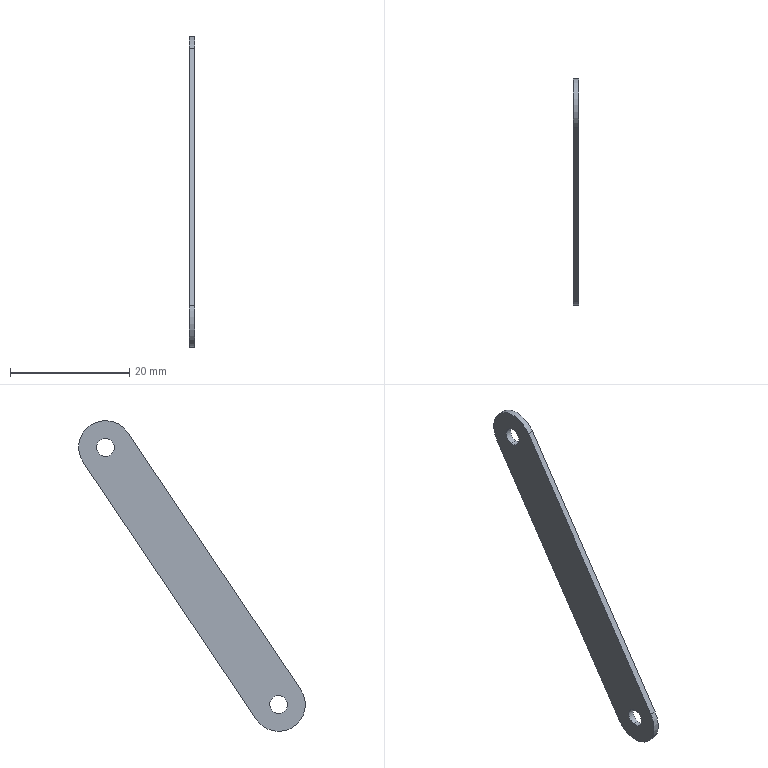Component | SolidWorks | Part12-2 | 1 solid | 11 faces | box 1 x 38.06 x 52.17 mm | volume 518 mm3 | cylinder 7 | plane 4 | commonest cylinder face diameters 3 x4 9 x3
build123d program:
from build123d import *

# Parameters (mm, degrees)
BOSS_EXTRUDE1_DEPTH = 1
BOSS_EXTRUDE2_START = -1
BOSS_EXTRUDE2_DEPTH = 1


with BuildPart() as part:
    # Sketch1 → Boss-Extrude1 (new body)
    with BuildSketch(Plane.XY):
        with BuildLine():
            Line((6.19, 34.803), (42.061, 72.502))
            ThreePointArc((42.061, 72.502), (48.423, 72.66), (48.581, 66.298))
            Line((48.581, 66.298), (12.71, 28.599))
            ThreePointArc((12.71, 28.599), (6.348, 28.441), (6.19, 34.803))
        make_face()
        with BuildLine():
            Line((8.363, 32.735), (44.235, 70.434))
            ThreePointArc((44.235, 70.434), (46.355, 70.487), (46.408, 68.366))
            Line((46.408, 68.366), (10.536, 30.667))
            ThreePointArc((10.536, 30.667), (8.416, 30.614), (8.363, 32.735))
        make_face(mode=Mode.SUBTRACT)
    extrude(amount=BOSS_EXTRUDE1_DEPTH)

    # Sketch2 → Boss-Extrude2 (add)
    with BuildSketch(Plane.XY.offset(1).offset(BOSS_EXTRUDE2_START)):
        with BuildLine():
            Line((10.536, 30.667), (46.408, 68.366))
            ThreePointArc((46.408, 68.366), (44.287, 68.314), (44.235, 70.434))
            Line((44.235, 70.434), (8.363, 32.735))
            ThreePointArc((8.363, 32.735), (10.484, 32.788), (10.536, 30.667))
        make_face()
    extrude(amount=BOSS_EXTRUDE2_DEPTH)


solid = part.part

# Placed as in the assembly
solid = solid.moved(Location((89.229, 6.521, -1.578), (12.475, -90, 0)))
STEP:
#1=COLOUR_RGB('',0.7922,0.8196,0.9333);
#2=FILL_AREA_STYLE_COLOUR('',#1);
#3=FILL_AREA_STYLE('',(#2));
#4=SURFACE_STYLE_FILL_AREA(#3);
#5=SURFACE_SIDE_STYLE('',(#4));
#6=SURFACE_STYLE_USAGE(.BOTH.,#5);
#7=PRESENTATION_STYLE_ASSIGNMENT((#6));
#8=CARTESIAN_POINT('',(3.474,2.552,2.213));
#9=VERTEX_POINT('',#8);
#10=CARTESIAN_POINT('',(3.474,2.526,2.328));
#11=VERTEX_POINT('',#10);
#12=CARTESIAN_POINT('',(3.474,2.539,2.27));
#13=DIRECTION('',(-1.,0.,0.));
#14=DIRECTION('',(0.,-0.216,0.9764));
#15=AXIS2_PLACEMENT_3D('',#12,#13,#14);
#16=CIRCLE('',#15,0.05906);
#17=EDGE_CURVE('',#9,#11,#16,.T.);
#18=ORIENTED_EDGE('',*,*,#17,.T.);
#19=CARTESIAN_POINT('',(3.513,2.526,2.328));
#20=VERTEX_POINT('',#19);
#21=CARTESIAN_POINT('',(3.474,2.526,2.328));
#22=DIRECTION('',(1.,-0.,-0.));
#23=VECTOR('',#22,39.37);
#24=LINE('',#21,#23);
#25=EDGE_CURVE('',#11,#20,#24,.T.);
#26=ORIENTED_EDGE('',*,*,#25,.T.);
#27=CARTESIAN_POINT('',(3.513,2.552,2.213));
#28=VERTEX_POINT('',#27);
#29=CARTESIAN_POINT('',(3.513,2.539,2.27));
#30=DIRECTION('',(-1.,0.,0.));
#31=DIRECTION('',(0.,-0.216,0.9764));
#32=AXIS2_PLACEMENT_3D('',#29,#30,#31);
#33=CIRCLE('',#32,0.05906);
#34=EDGE_CURVE('',#28,#20,#33,.T.);
#35=ORIENTED_EDGE('',*,*,#34,.F.);
#36=CARTESIAN_POINT('',(3.474,2.552,2.213));
#37=DIRECTION('',(1.,-0.,-0.));
#38=VECTOR('',#37,39.37);
#39=LINE('',#36,#38);
#40=EDGE_CURVE('',#9,#28,#39,.T.);
#41=ORIENTED_EDGE('',*,*,#40,.F.);
#42=EDGE_LOOP('',(#18,#26,#35,#41));
#43=FACE_OUTER_BOUND('',#42,.T.);
#44=CARTESIAN_POINT('',(3.474,2.539,2.27));
#45=DIRECTION('',(1.,-0.,-0.));
#46=DIRECTION('',(0.,0.216,-0.9764));
#47=AXIS2_PLACEMENT_3D('',#44,#45,#46);
#48=CYLINDRICAL_SURFACE('',#47,0.05906);
#49=ADVANCED_FACE('',(#43),#48,.F.);
#50=CARTESIAN_POINT('',(3.474,1.408,0.5131));
#51=VERTEX_POINT('',#50);
#52=CARTESIAN_POINT('',(3.474,1.382,0.6284));
#53=VERTEX_POINT('',#52);
#54=CARTESIAN_POINT('',(3.474,1.395,0.5707));
#55=DIRECTION('',(-1.,0.,0.));
#56=DIRECTION('',(0.,-0.216,0.9764));
#57=AXIS2_PLACEMENT_3D('',#54,#55,#56);
#58=CIRCLE('',#57,0.05906);
#59=EDGE_CURVE('',#51,#53,#58,.T.);
#60=ORIENTED_EDGE('',*,*,#59,.T.);
#61=CARTESIAN_POINT('',(3.513,1.382,0.6284));
#62=VERTEX_POINT('',#61);
#63=CARTESIAN_POINT('',(3.474,1.382,0.6284));
#64=DIRECTION('',(1.,-0.,-0.));
#65=VECTOR('',#64,39.37);
#66=LINE('',#63,#65);
#67=EDGE_CURVE('',#53,#62,#66,.T.);
#68=ORIENTED_EDGE('',*,*,#67,.T.);
#69=CARTESIAN_POINT('',(3.513,1.408,0.5131));
#70=VERTEX_POINT('',#69);
#71=CARTESIAN_POINT('',(3.513,1.395,0.5707));
#72=DIRECTION('',(-1.,0.,0.));
#73=DIRECTION('',(0.,-0.216,0.9764));
#74=AXIS2_PLACEMENT_3D('',#71,#72,#73);
#75=CIRCLE('',#74,0.05906);
#76=EDGE_CURVE('',#70,#62,#75,.T.);
#77=ORIENTED_EDGE('',*,*,#76,.F.);
#78=CARTESIAN_POINT('',(3.474,1.408,0.5131));
#79=DIRECTION('',(1.,-0.,-0.));
#80=VECTOR('',#79,39.37);
#81=LINE('',#78,#80);
#82=EDGE_CURVE('',#51,#70,#81,.T.);
#83=ORIENTED_EDGE('',*,*,#82,.F.);
#84=EDGE_LOOP('',(#60,#68,#77,#83));
#85=FACE_OUTER_BOUND('',#84,.T.);
#86=CARTESIAN_POINT('',(3.474,1.395,0.5707));
#87=DIRECTION('',(1.,-0.,-0.));
#88=DIRECTION('',(0.,0.216,-0.9764));
#89=AXIS2_PLACEMENT_3D('',#86,#87,#88);
#90=CYLINDRICAL_SURFACE('',#89,0.05906);
#91=ADVANCED_FACE('',(#85),#90,.F.);
#92=CARTESIAN_POINT('',(3.474,1.433,0.3978));
#93=VERTEX_POINT('',#92);
#94=CARTESIAN_POINT('',(3.474,1.248,0.6697));
#95=VERTEX_POINT('',#94);
#96=CARTESIAN_POINT('',(3.474,1.395,0.5707));
#97=DIRECTION('',(-1.,0.,0.));
#98=DIRECTION('',(0.,-0.216,0.9764));
#99=AXIS2_PLACEMENT_3D('',#96,#97,#98);
#100=CIRCLE('',#99,0.1772);
#101=EDGE_CURVE('',#93,#95,#100,.T.);
#102=ORIENTED_EDGE('',*,*,#101,.F.);
#103=CARTESIAN_POINT('',(3.513,1.433,0.3978));
#104=VERTEX_POINT('',#103);
#105=CARTESIAN_POINT('',(3.474,1.433,0.3978));
#106=DIRECTION('',(1.,-0.,-0.));
#107=VECTOR('',#106,39.37);
#108=LINE('',#105,#107);
#109=EDGE_CURVE('',#93,#104,#108,.T.);
#110=ORIENTED_EDGE('',*,*,#109,.T.);
#111=CARTESIAN_POINT('',(3.513,1.248,0.6697));
#112=VERTEX_POINT('',#111);
#113=CARTESIAN_POINT('',(3.513,1.395,0.5707));
#114=DIRECTION('',(-1.,0.,0.));
#115=DIRECTION('',(0.,-0.216,0.9764));
#116=AXIS2_PLACEMENT_3D('',#113,#114,#115);
#117=CIRCLE('',#116,0.1772);
#118=EDGE_CURVE('',#104,#112,#117,.T.);
#119=ORIENTED_EDGE('',*,*,#118,.T.);
#120=CARTESIAN_POINT('',(3.474,1.248,0.6697));
#121=DIRECTION('',(1.,-0.,-0.));
#122=VECTOR('',#121,39.37);
#123=LINE('',#120,#122);
#124=EDGE_CURVE('',#95,#112,#123,.T.);
#125=ORIENTED_EDGE('',*,*,#124,.F.);
#126=EDGE_LOOP('',(#102,#110,#119,#125));
#127=FACE_OUTER_BOUND('',#126,.T.);
#128=CARTESIAN_POINT('',(3.474,1.395,0.5707));
#129=DIRECTION('',(1.,-0.,-0.));
#130=DIRECTION('',(0.,0.216,-0.9764));
#131=AXIS2_PLACEMENT_3D('',#128,#129,#130);
#132=CYLINDRICAL_SURFACE('',#131,0.1772);
#133=ADVANCED_FACE('',(#127),#132,.T.);
#134=ORIENTED_EDGE('',*,*,#17,.F.);
#135=CARTESIAN_POINT('',(3.474,2.539,2.27));
#136=DIRECTION('',(-1.,0.,0.));
#137=DIRECTION('',(0.,-0.216,0.9764));
#138=AXIS2_PLACEMENT_3D('',#135,#136,#137);
#139=CIRCLE('',#138,0.05906);
#140=EDGE_CURVE('',#11,#9,#139,.T.);
#141=ORIENTED_EDGE('',*,*,#140,.F.);
#142=EDGE_LOOP('',(#134,#141));
#143=FACE_BOUND('',#142,.T.);
#144=CARTESIAN_POINT('',(3.474,1.542,0.4718));
#145=VERTEX_POINT('',#144);
#146=CARTESIAN_POINT('',(3.474,1.395,0.5707));
#147=DIRECTION('',(-1.,0.,0.));
#148=DIRECTION('',(0.,-0.216,0.9764));
#149=AXIS2_PLACEMENT_3D('',#146,#147,#148);
#150=CIRCLE('',#149,0.1772);
#151=EDGE_CURVE('',#145,#93,#150,.T.);
#152=ORIENTED_EDGE('',*,*,#151,.T.);
#153=ORIENTED_EDGE('',*,*,#101,.T.);
#154=CARTESIAN_POINT('',(3.474,2.392,2.369));
#155=VERTEX_POINT('',#154);
#156=CARTESIAN_POINT('',(3.474,1.248,0.6697));
#157=DIRECTION('',(0.,0.5584,0.8295));
#158=VECTOR('',#157,39.37);
#159=LINE('',#156,#158);
#160=EDGE_CURVE('',#95,#155,#159,.T.);
#161=ORIENTED_EDGE('',*,*,#160,.T.);
#162=CARTESIAN_POINT('',(3.474,2.686,2.171));
#163=VERTEX_POINT('',#162);
#164=CARTESIAN_POINT('',(3.474,2.539,2.27));
#165=DIRECTION('',(-1.,0.,0.));
#166=DIRECTION('',(0.,-0.216,0.9764));
#167=AXIS2_PLACEMENT_3D('',#164,#165,#166);
#168=CIRCLE('',#167,0.1772);
#169=EDGE_CURVE('',#155,#163,#168,.T.);
#170=ORIENTED_EDGE('',*,*,#169,.T.);
#171=CARTESIAN_POINT('',(3.474,1.542,0.4718));
#172=DIRECTION('',(-0.,-0.5584,-0.8295));
#173=VECTOR('',#172,39.37);
#174=LINE('',#171,#173);
#175=EDGE_CURVE('',#163,#145,#174,.T.);
#176=ORIENTED_EDGE('',*,*,#175,.T.);
#177=EDGE_LOOP('',(#152,#153,#161,#170,#176));
#178=FACE_OUTER_BOUND('',#177,.T.);
#179=ORIENTED_EDGE('',*,*,#59,.F.);
#180=CARTESIAN_POINT('',(3.474,1.395,0.5707));
#181=DIRECTION('',(-1.,0.,0.));
#182=DIRECTION('',(0.,-0.216,0.9764));
#183=AXIS2_PLACEMENT_3D('',#180,#181,#182);
#184=CIRCLE('',#183,0.05906);
#185=EDGE_CURVE('',#53,#51,#184,.T.);
#186=ORIENTED_EDGE('',*,*,#185,.F.);
#187=EDGE_LOOP('',(#179,#186));
#188=FACE_BOUND('',#187,.T.);
#189=CARTESIAN_POINT('',(3.474,1.395,0.5707));
#190=DIRECTION('',(-1.,0.,0.));
#191=DIRECTION('',(0.,-0.216,0.9764));
#192=AXIS2_PLACEMENT_3D('',#189,#190,#191);
#193=PLANE('',#192);
#194=ADVANCED_FACE('',(#143,#178,#188),#193,.T.);
#195=ORIENTED_EDGE('',*,*,#34,.T.);
#196=CARTESIAN_POINT('',(3.513,2.539,2.27));
#197=DIRECTION('',(-1.,0.,0.));
#198=DIRECTION('',(0.,-0.216,0.9764));
#199=AXIS2_PLACEMENT_3D('',#196,#197,#198);
#200=CIRCLE('',#199,0.05906);
#201=EDGE_CURVE('',#20,#28,#200,.T.);
#202=ORIENTED_EDGE('',*,*,#201,.T.);
#203=EDGE_LOOP('',(#195,#202));
#204=FACE_BOUND('',#203,.T.);
#205=CARTESIAN_POINT('',(3.513,1.542,0.4718));
#206=VERTEX_POINT('',#205);
#207=CARTESIAN_POINT('',(3.513,1.395,0.5707));
#208=DIRECTION('',(-1.,0.,0.));
#209=DIRECTION('',(0.,-0.216,0.9764));
#210=AXIS2_PLACEMENT_3D('',#207,#208,#209);
#211=CIRCLE('',#210,0.1772);
#212=EDGE_CURVE('',#206,#104,#211,.T.);
#213=ORIENTED_EDGE('',*,*,#212,.F.);
#214=CARTESIAN_POINT('',(3.513,2.686,2.171));
#215=VERTEX_POINT('',#214);
#216=CARTESIAN_POINT('',(3.513,1.542,0.4718));
#217=DIRECTION('',(-0.,-0.5584,-0.8295));
#218=VECTOR('',#217,39.37);
#219=LINE('',#216,#218);
#220=EDGE_CURVE('',#215,#206,#219,.T.);
#221=ORIENTED_EDGE('',*,*,#220,.F.);
#222=CARTESIAN_POINT('',(3.513,2.392,2.369));
#223=VERTEX_POINT('',#222);
#224=CARTESIAN_POINT('',(3.513,2.539,2.27));
#225=DIRECTION('',(-1.,0.,0.));
#226=DIRECTION('',(0.,-0.216,0.9764));
#227=AXIS2_PLACEMENT_3D('',#224,#225,#226);
#228=CIRCLE('',#227,0.1772);
#229=EDGE_CURVE('',#223,#215,#228,.T.);
#230=ORIENTED_EDGE('',*,*,#229,.F.);
#231=CARTESIAN_POINT('',(3.513,1.248,0.6697));
#232=DIRECTION('',(0.,0.5584,0.8295));
#233=VECTOR('',#232,39.37);
#234=LINE('',#231,#233);
#235=EDGE_CURVE('',#112,#223,#234,.T.);
#236=ORIENTED_EDGE('',*,*,#235,.F.);
#237=ORIENTED_EDGE('',*,*,#118,.F.);
#238=EDGE_LOOP('',(#213,#221,#230,#236,#237));
#239=FACE_OUTER_BOUND('',#238,.T.);
#240=ORIENTED_EDGE('',*,*,#76,.T.);
#241=CARTESIAN_POINT('',(3.513,1.395,0.5707));
#242=DIRECTION('',(-1.,0.,0.));
#243=DIRECTION('',(0.,-0.216,0.9764));
#244=AXIS2_PLACEMENT_3D('',#241,#242,#243);
#245=CIRCLE('',#244,0.05906);
#246=EDGE_CURVE('',#62,#70,#245,.T.);
#247=ORIENTED_EDGE('',*,*,#246,.T.);
#248=EDGE_LOOP('',(#240,#247));
#249=FACE_BOUND('',#248,.T.);
#250=CARTESIAN_POINT('',(3.513,1.395,0.5707));
#251=DIRECTION('',(-1.,0.,0.));
#252=DIRECTION('',(0.,-0.216,0.9764));
#253=AXIS2_PLACEMENT_3D('',#250,#251,#252);
#254=PLANE('',#253);
#255=ADVANCED_FACE('',(#204,#239,#249),#254,.F.);
#256=ORIENTED_EDGE('',*,*,#109,.F.);
#257=ORIENTED_EDGE('',*,*,#151,.F.);
#258=CARTESIAN_POINT('',(3.474,1.542,0.4718));
#259=DIRECTION('',(1.,-0.,-0.));
#260=VECTOR('',#259,39.37);
#261=LINE('',#258,#260);
#262=EDGE_CURVE('',#145,#206,#261,.T.);
#263=ORIENTED_EDGE('',*,*,#262,.T.);
#264=ORIENTED_EDGE('',*,*,#212,.T.);
#265=EDGE_LOOP('',(#256,#257,#263,#264));
#266=FACE_OUTER_BOUND('',#265,.T.);
#267=CARTESIAN_POINT('',(3.474,1.395,0.5707));
#268=DIRECTION('',(1.,-0.,-0.));
#269=DIRECTION('',(0.,0.216,-0.9764));
#270=AXIS2_PLACEMENT_3D('',#267,#268,#269);
#271=CYLINDRICAL_SURFACE('',#270,0.1772);
#272=ADVANCED_FACE('',(#266),#271,.T.);
#273=ORIENTED_EDGE('',*,*,#235,.T.);
#274=CARTESIAN_POINT('',(3.474,2.392,2.369));
#275=DIRECTION('',(1.,-0.,-0.));
#276=VECTOR('',#275,39.37);
#277=LINE('',#274,#276);
#278=EDGE_CURVE('',#155,#223,#277,.T.);
#279=ORIENTED_EDGE('',*,*,#278,.F.);
#280=ORIENTED_EDGE('',*,*,#160,.F.);
#281=ORIENTED_EDGE('',*,*,#124,.T.);
#282=EDGE_LOOP('',(#273,#279,#280,#281));
#283=FACE_OUTER_BOUND('',#282,.T.);
#284=CARTESIAN_POINT('',(3.474,1.248,0.6697));
#285=DIRECTION('',(0.,0.8295,-0.5584));
#286=DIRECTION('',(-0.,-0.5584,-0.8295));
#287=AXIS2_PLACEMENT_3D('',#284,#285,#286);
#288=PLANE('',#287);
#289=ADVANCED_FACE('',(#283),#288,.F.);
#290=ORIENTED_EDGE('',*,*,#229,.T.);
#291=CARTESIAN_POINT('',(3.474,2.686,2.171));
#292=DIRECTION('',(1.,-0.,-0.));
#293=VECTOR('',#292,39.37);
#294=LINE('',#291,#293);
#295=EDGE_CURVE('',#163,#215,#294,.T.);
#296=ORIENTED_EDGE('',*,*,#295,.F.);
#297=ORIENTED_EDGE('',*,*,#169,.F.);
#298=ORIENTED_EDGE('',*,*,#278,.T.);
#299=EDGE_LOOP('',(#290,#296,#297,#298));
#300=FACE_OUTER_BOUND('',#299,.T.);
#301=CARTESIAN_POINT('',(3.474,2.539,2.27));
#302=DIRECTION('',(1.,-0.,-0.));
#303=DIRECTION('',(0.,0.216,-0.9764));
#304=AXIS2_PLACEMENT_3D('',#301,#302,#303);
#305=CYLINDRICAL_SURFACE('',#304,0.1772);
#306=ADVANCED_FACE('',(#300),#305,.T.);
#307=ORIENTED_EDGE('',*,*,#220,.T.);
#308=ORIENTED_EDGE('',*,*,#262,.F.);
#309=ORIENTED_EDGE('',*,*,#175,.F.);
#310=ORIENTED_EDGE('',*,*,#295,.T.);
#311=EDGE_LOOP('',(#307,#308,#309,#310));
#312=FACE_OUTER_BOUND('',#311,.T.);
#313=CARTESIAN_POINT('',(3.474,1.542,0.4718));
#314=DIRECTION('',(-0.,-0.8295,0.5584));
#315=DIRECTION('',(0.,0.5584,0.8295));
#316=AXIS2_PLACEMENT_3D('',#313,#314,#315);
#317=PLANE('',#316);
#318=ADVANCED_FACE('',(#312),#317,.F.);
#319=ORIENTED_EDGE('',*,*,#67,.F.);
#320=ORIENTED_EDGE('',*,*,#185,.T.);
#321=ORIENTED_EDGE('',*,*,#82,.T.);
#322=ORIENTED_EDGE('',*,*,#246,.F.);
#323=EDGE_LOOP('',(#319,#320,#321,#322));
#324=FACE_OUTER_BOUND('',#323,.T.);
#325=CARTESIAN_POINT('',(3.474,1.395,0.5707));
#326=DIRECTION('',(1.,-0.,-0.));
#327=DIRECTION('',(0.,0.216,-0.9764));
#328=AXIS2_PLACEMENT_3D('',#325,#326,#327);
#329=CYLINDRICAL_SURFACE('',#328,0.05906);
#330=ADVANCED_FACE('',(#324),#329,.F.);
#331=ORIENTED_EDGE('',*,*,#25,.F.);
#332=ORIENTED_EDGE('',*,*,#140,.T.);
#333=ORIENTED_EDGE('',*,*,#40,.T.);
#334=ORIENTED_EDGE('',*,*,#201,.F.);
#335=EDGE_LOOP('',(#331,#332,#333,#334));
#336=FACE_OUTER_BOUND('',#335,.T.);
#337=CARTESIAN_POINT('',(3.474,2.539,2.27));
#338=DIRECTION('',(1.,-0.,-0.));
#339=DIRECTION('',(0.,0.216,-0.9764));
#340=AXIS2_PLACEMENT_3D('',#337,#338,#339);
#341=CYLINDRICAL_SURFACE('',#340,0.05906);
#342=ADVANCED_FACE('',(#336),#341,.F.);
#343=CLOSED_SHELL('',(#49,#91,#133,#194,#255,#272,#289,#306,#318,#330,#342));
#344=MANIFOLD_SOLID_BREP('',#343);
#345=STYLED_ITEM('',(#7),#344);
#346=(LENGTH_UNIT()NAMED_UNIT(*)SI_UNIT($,.METRE.));
#347=LENGTH_MEASURE_WITH_UNIT(LENGTH_MEASURE(0.0254),#346);
#348=DIMENSIONAL_EXPONENTS(1.,0.,0.,0.,0.,0.,0.);
#349=(CONVERSION_BASED_UNIT('',#347)LENGTH_UNIT()NAMED_UNIT(#348));
#350=UNCERTAINTY_MEASURE_WITH_UNIT(LENGTH_MEASURE(0.00001),#349,'','');
#351=(NAMED_UNIT(*)PLANE_ANGLE_UNIT()SI_UNIT($,.RADIAN.));
#352=(NAMED_UNIT(*)SI_UNIT($,.STERADIAN.)SOLID_ANGLE_UNIT());
#353=(GEOMETRIC_REPRESENTATION_CONTEXT(3)GLOBAL_UNCERTAINTY_ASSIGNED_CONTEXT((#350))GLOBAL_UNIT_ASSIGNED_CONTEXT((#349,#351,#352))REPRESENTATION_CONTEXT('',''));
#354=MECHANICAL_DESIGN_GEOMETRIC_PRESENTATION_REPRESENTATION('',(#345),#353);
#355=PRESENTATION_LAYER_ASSIGNMENT('','',(#345));
#356=CARTESIAN_POINT('',(0.,0.,0.));
#357=DIRECTION('',(0.,0.,1.));
#358=DIRECTION('',(1.,0.,0.));
#359=AXIS2_PLACEMENT_3D('',#356,#357,#358);
#360=(LENGTH_UNIT()NAMED_UNIT(*)SI_UNIT($,.METRE.));
#361=LENGTH_MEASURE_WITH_UNIT(LENGTH_MEASURE(0.0254),#360);
#362=DIMENSIONAL_EXPONENTS(1.,0.,0.,0.,0.,0.,0.);
#363=(CONVERSION_BASED_UNIT('',#361)LENGTH_UNIT()NAMED_UNIT(#362));
#364=UNCERTAINTY_MEASURE_WITH_UNIT(LENGTH_MEASURE(0.00001),#363,'','');
#365=(NAMED_UNIT(*)PLANE_ANGLE_UNIT()SI_UNIT($,.RADIAN.));
#366=(NAMED_UNIT(*)SI_UNIT($,.STERADIAN.)SOLID_ANGLE_UNIT());
#367=(GEOMETRIC_REPRESENTATION_CONTEXT(3)GLOBAL_UNCERTAINTY_ASSIGNED_CONTEXT((#364))GLOBAL_UNIT_ASSIGNED_CONTEXT((#363,#365,#366))REPRESENTATION_CONTEXT('',''));
#368=ADVANCED_BREP_SHAPE_REPRESENTATION('',(#344,#359),#367);